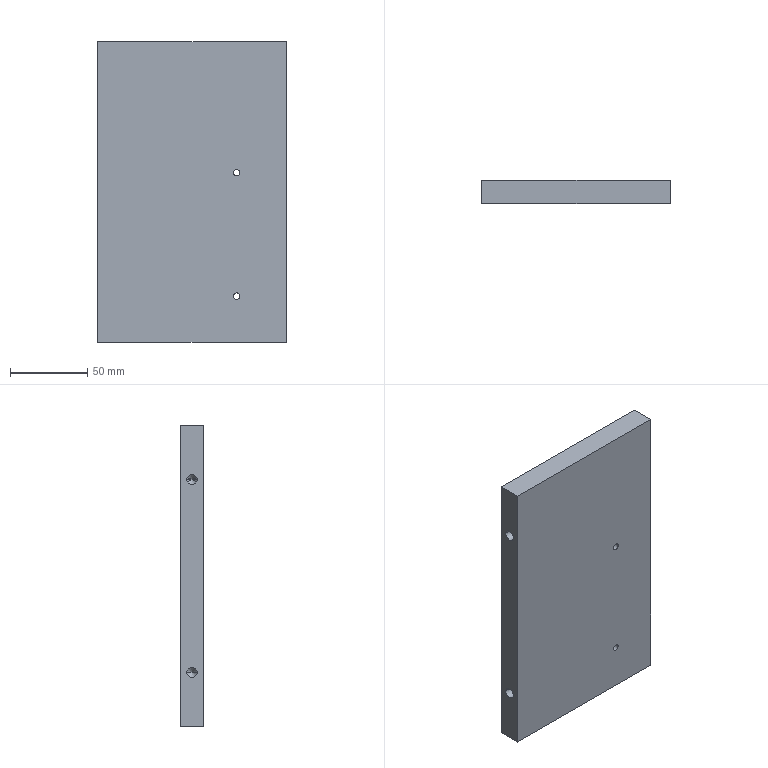Component | SolidWorks | InnerBagLiftingCylinderFixingPlate-1 | 1 solid | 26 faces | box 122 x 15 x 195 mm | volume 354555 mm3 | cylinder 12 | cone 8 | plane 6 | commonest cylinder face diameters 4.2 x8 6.8 x4
build123d program:
from build123d import *

# Parameters (mm, degrees)
SKETCH1_W             = 122
SKETCH1_H             = 195
BOSS_EXTRUDE1_DEPTH   = 7.5
M8_TAPPED_HOLE1_D     = 6.8
M8_TAPPED_HOLE1_DEPTH = 19.75
M8_TAPPED_HOLE1_TIP   = 3.4
M5_TAPPED_HOLE1_D     = 4.2
M5_TAPPED_HOLE2_D     = 4.2
M5_TAPPED_HOLE2_DEPTH = 12.4
M5_TAPPED_HOLE2_TIP   = 2.1


with BuildPart() as part:
    # Sketch1 → Boss-Extrude1 (new, symmetric)
    with BuildSketch(Plane.XY):
        with Locations((61, 97.5)):
            Rectangle(SKETCH1_W, SKETCH1_H)
    extrude(amount=BOSS_EXTRUDE1_DEPTH, both=True)

    # M8 Tapped Hole1
    with Locations(Plane(origin=(0, 160, 0), x_dir=(0, 0, -1), z_dir=(-1, 0, 0))):
        with Locations((0, 0), (0, 125)):
            Hole(M8_TAPPED_HOLE1_D / 2, depth=M8_TAPPED_HOLE1_DEPTH)
            with Locations((0, 0, -(M8_TAPPED_HOLE1_DEPTH + M8_TAPPED_HOLE1_TIP / 2))):  # 90° drill point
                Cone(0, M8_TAPPED_HOLE1_D / 2, M8_TAPPED_HOLE1_TIP, mode=Mode.SUBTRACT)

    # M5 Tapped Hole1 (through all)
    with Locations(Plane(origin=(90, 110, 7.5), x_dir=(1, 0, 0), z_dir=(0, 0, 1))):
        with Locations((0, 0), (0, -80)):
            Hole(M5_TAPPED_HOLE1_D / 2)

    # M5 Tapped Hole2
    with Locations(Plane(origin=(0, 0, 0), x_dir=(-1, 0, 0), z_dir=(0, -1, 0))):
        with Locations((-76, 0), (-104, 0)):
            Hole(M5_TAPPED_HOLE2_D / 2, depth=M5_TAPPED_HOLE2_DEPTH)
            with Locations((0, 0, -(M5_TAPPED_HOLE2_DEPTH + M5_TAPPED_HOLE2_TIP / 2))):  # 90° drill point
                Cone(0, M5_TAPPED_HOLE2_D / 2, M5_TAPPED_HOLE2_TIP, mode=Mode.SUBTRACT)


solid = part.part

# Placed as in the assembly
solid = solid.moved(Location((-22.646, -26.568, 148.933), (90, 0, 0)))
STEP:
#1=COLOUR_RGB('',0.7922,0.8196,0.9333);
#2=FILL_AREA_STYLE_COLOUR('',#1);
#3=FILL_AREA_STYLE('',(#2));
#4=SURFACE_STYLE_FILL_AREA(#3);
#5=SURFACE_SIDE_STYLE('',(#4));
#6=SURFACE_STYLE_USAGE(.BOTH.,#5);
#7=PRESENTATION_STYLE_ASSIGNMENT((#6));
#8=CARTESIAN_POINT('',(2.101,-1.129,6.352));
#9=VERTEX_POINT('',#8);
#10=CARTESIAN_POINT('',(2.101,-0.9633,6.352));
#11=VERTEX_POINT('',#10);
#12=CARTESIAN_POINT('',(2.101,-1.046,6.352));
#13=DIRECTION('',(0.,0.,-1.));
#14=DIRECTION('',(0.,1.,0.));
#15=AXIS2_PLACEMENT_3D('',#12,#13,#14);
#16=CIRCLE('',#15,0.08268);
#17=EDGE_CURVE('',#9,#11,#16,.T.);
#18=ORIENTED_EDGE('',*,*,#17,.F.);
#19=CARTESIAN_POINT('',(2.101,-1.129,5.863));
#20=VERTEX_POINT('',#19);
#21=CARTESIAN_POINT('',(2.101,-1.129,5.863));
#22=DIRECTION('',(0.,0.,-1.));
#23=VECTOR('',#22,39.37);
#24=LINE('',#21,#23);
#25=EDGE_CURVE('',#9,#20,#24,.T.);
#26=ORIENTED_EDGE('',*,*,#25,.T.);
#27=CARTESIAN_POINT('',(2.101,-0.9633,5.863));
#28=VERTEX_POINT('',#27);
#29=CARTESIAN_POINT('',(2.101,-1.046,5.863));
#30=DIRECTION('',(0.,0.,-1.));
#31=DIRECTION('',(0.,1.,0.));
#32=AXIS2_PLACEMENT_3D('',#29,#30,#31);
#33=CIRCLE('',#32,0.08268);
#34=EDGE_CURVE('',#20,#28,#33,.T.);
#35=ORIENTED_EDGE('',*,*,#34,.T.);
#36=CARTESIAN_POINT('',(2.101,-0.9633,5.863));
#37=DIRECTION('',(0.,0.,-1.));
#38=VECTOR('',#37,39.37);
#39=LINE('',#36,#38);
#40=EDGE_CURVE('',#11,#28,#39,.T.);
#41=ORIENTED_EDGE('',*,*,#40,.F.);
#42=EDGE_LOOP('',(#18,#26,#35,#41));
#43=FACE_OUTER_BOUND('',#42,.T.);
#44=CARTESIAN_POINT('',(2.101,-1.046,5.863));
#45=DIRECTION('',(0.,0.,-1.));
#46=DIRECTION('',(0.,1.,0.));
#47=AXIS2_PLACEMENT_3D('',#44,#45,#46);
#48=CYLINDRICAL_SURFACE('',#47,0.08268);
#49=ADVANCED_FACE('',(#43),#48,.F.);
#50=CARTESIAN_POINT('',(2.101,-1.046,6.434));
#51=VERTEX_POINT('',#50);
#52=CARTESIAN_POINT('',(2.101,-0.9633,6.352));
#53=DIRECTION('',(0.,0.7071,-0.7071));
#54=VECTOR('',#53,39.37);
#55=LINE('',#52,#54);
#56=EDGE_CURVE('',#51,#11,#55,.T.);
#57=ORIENTED_EDGE('',*,*,#56,.F.);
#58=CARTESIAN_POINT('',(2.101,-1.129,6.352));
#59=DIRECTION('',(0.,-0.7071,-0.7071));
#60=VECTOR('',#59,39.37);
#61=LINE('',#58,#60);
#62=EDGE_CURVE('',#51,#9,#61,.T.);
#63=ORIENTED_EDGE('',*,*,#62,.T.);
#64=ORIENTED_EDGE('',*,*,#17,.T.);
#65=EDGE_LOOP('',(#57,#63,#64));
#66=FACE_OUTER_BOUND('',#65,.T.);
#67=CARTESIAN_POINT('',(2.101,-1.046,6.352));
#68=DIRECTION('',(0.,0.,-1.));
#69=DIRECTION('',(0.,1.,0.));
#70=AXIS2_PLACEMENT_3D('',#67,#68,#69);
#71=CONICAL_SURFACE('',#70,0.08268,0.7854);
#72=ADVANCED_FACE('',(#66),#71,.F.);
#73=CARTESIAN_POINT('',(3.203,-1.129,6.352));
#74=VERTEX_POINT('',#73);
#75=CARTESIAN_POINT('',(3.203,-0.9633,6.352));
#76=VERTEX_POINT('',#75);
#77=CARTESIAN_POINT('',(3.203,-1.046,6.352));
#78=DIRECTION('',(0.,0.,-1.));
#79=DIRECTION('',(0.,1.,0.));
#80=AXIS2_PLACEMENT_3D('',#77,#78,#79);
#81=CIRCLE('',#80,0.08268);
#82=EDGE_CURVE('',#74,#76,#81,.T.);
#83=ORIENTED_EDGE('',*,*,#82,.F.);
#84=CARTESIAN_POINT('',(3.203,-1.129,5.863));
#85=VERTEX_POINT('',#84);
#86=CARTESIAN_POINT('',(3.203,-1.129,5.863));
#87=DIRECTION('',(0.,0.,-1.));
#88=VECTOR('',#87,39.37);
#89=LINE('',#86,#88);
#90=EDGE_CURVE('',#74,#85,#89,.T.);
#91=ORIENTED_EDGE('',*,*,#90,.T.);
#92=CARTESIAN_POINT('',(3.203,-0.9633,5.863));
#93=VERTEX_POINT('',#92);
#94=CARTESIAN_POINT('',(3.203,-1.046,5.863));
#95=DIRECTION('',(0.,0.,-1.));
#96=DIRECTION('',(0.,1.,0.));
#97=AXIS2_PLACEMENT_3D('',#94,#95,#96);
#98=CIRCLE('',#97,0.08268);
#99=EDGE_CURVE('',#85,#93,#98,.T.);
#100=ORIENTED_EDGE('',*,*,#99,.T.);
#101=CARTESIAN_POINT('',(3.203,-0.9633,5.863));
#102=DIRECTION('',(0.,0.,-1.));
#103=VECTOR('',#102,39.37);
#104=LINE('',#101,#103);
#105=EDGE_CURVE('',#76,#93,#104,.T.);
#106=ORIENTED_EDGE('',*,*,#105,.F.);
#107=EDGE_LOOP('',(#83,#91,#100,#106));
#108=FACE_OUTER_BOUND('',#107,.T.);
#109=CARTESIAN_POINT('',(3.203,-1.046,5.863));
#110=DIRECTION('',(0.,0.,-1.));
#111=DIRECTION('',(0.,1.,0.));
#112=AXIS2_PLACEMENT_3D('',#109,#110,#111);
#113=CYLINDRICAL_SURFACE('',#112,0.08268);
#114=ADVANCED_FACE('',(#108),#113,.F.);
#115=CARTESIAN_POINT('',(3.203,-1.046,6.434));
#116=VERTEX_POINT('',#115);
#117=CARTESIAN_POINT('',(3.203,-0.9633,6.352));
#118=DIRECTION('',(0.,0.7071,-0.7071));
#119=VECTOR('',#118,39.37);
#120=LINE('',#117,#119);
#121=EDGE_CURVE('',#116,#76,#120,.T.);
#122=ORIENTED_EDGE('',*,*,#121,.F.);
#123=CARTESIAN_POINT('',(3.203,-1.129,6.352));
#124=DIRECTION('',(0.,-0.7071,-0.7071));
#125=VECTOR('',#124,39.37);
#126=LINE('',#123,#125);
#127=EDGE_CURVE('',#116,#74,#126,.T.);
#128=ORIENTED_EDGE('',*,*,#127,.T.);
#129=ORIENTED_EDGE('',*,*,#82,.T.);
#130=EDGE_LOOP('',(#122,#128,#129));
#131=FACE_OUTER_BOUND('',#130,.T.);
#132=CARTESIAN_POINT('',(3.203,-1.046,6.352));
#133=DIRECTION('',(0.,0.,-1.));
#134=DIRECTION('',(0.,1.,0.));
#135=AXIS2_PLACEMENT_3D('',#132,#133,#134);
#136=CONICAL_SURFACE('',#135,0.08268,0.7854);
#137=ADVANCED_FACE('',(#131),#136,.F.);
#138=CARTESIAN_POINT('',(2.569,-0.7507,10.194));
#139=VERTEX_POINT('',#138);
#140=CARTESIAN_POINT('',(2.734,-0.7507,10.194));
#141=VERTEX_POINT('',#140);
#142=CARTESIAN_POINT('',(2.652,-0.7507,10.194));
#143=DIRECTION('',(0.,-1.,0.));
#144=DIRECTION('',(1.,0.,0.));
#145=AXIS2_PLACEMENT_3D('',#142,#143,#144);
#146=CIRCLE('',#145,0.08268);
#147=EDGE_CURVE('',#139,#141,#146,.T.);
#148=ORIENTED_EDGE('',*,*,#147,.F.);
#149=CARTESIAN_POINT('',(2.569,-1.341,10.194));
#150=VERTEX_POINT('',#149);
#151=CARTESIAN_POINT('',(2.569,-1.341,10.194));
#152=DIRECTION('',(0.,-1.,0.));
#153=VECTOR('',#152,39.37);
#154=LINE('',#151,#153);
#155=EDGE_CURVE('',#139,#150,#154,.T.);
#156=ORIENTED_EDGE('',*,*,#155,.T.);
#157=CARTESIAN_POINT('',(2.734,-1.341,10.194));
#158=VERTEX_POINT('',#157);
#159=CARTESIAN_POINT('',(2.652,-1.341,10.194));
#160=DIRECTION('',(0.,-1.,0.));
#161=DIRECTION('',(1.,0.,0.));
#162=AXIS2_PLACEMENT_3D('',#159,#160,#161);
#163=CIRCLE('',#162,0.08268);
#164=EDGE_CURVE('',#150,#158,#163,.T.);
#165=ORIENTED_EDGE('',*,*,#164,.T.);
#166=CARTESIAN_POINT('',(2.734,-1.341,10.194));
#167=DIRECTION('',(0.,-1.,0.));
#168=VECTOR('',#167,39.37);
#169=LINE('',#166,#168);
#170=EDGE_CURVE('',#141,#158,#169,.T.);
#171=ORIENTED_EDGE('',*,*,#170,.F.);
#172=EDGE_LOOP('',(#148,#156,#165,#171));
#173=FACE_OUTER_BOUND('',#172,.T.);
#174=CARTESIAN_POINT('',(2.652,-1.341,10.194));
#175=DIRECTION('',(0.,-1.,0.));
#176=DIRECTION('',(1.,0.,0.));
#177=AXIS2_PLACEMENT_3D('',#174,#175,#176);
#178=CYLINDRICAL_SURFACE('',#177,0.08268);
#179=ADVANCED_FACE('',(#173),#178,.F.);
#180=CARTESIAN_POINT('',(2.569,-0.7507,7.045));
#181=VERTEX_POINT('',#180);
#182=CARTESIAN_POINT('',(2.734,-0.7507,7.045));
#183=VERTEX_POINT('',#182);
#184=CARTESIAN_POINT('',(2.652,-0.7507,7.045));
#185=DIRECTION('',(0.,-1.,0.));
#186=DIRECTION('',(1.,0.,0.));
#187=AXIS2_PLACEMENT_3D('',#184,#185,#186);
#188=CIRCLE('',#187,0.08268);
#189=EDGE_CURVE('',#181,#183,#188,.T.);
#190=ORIENTED_EDGE('',*,*,#189,.F.);
#191=CARTESIAN_POINT('',(2.569,-1.341,7.045));
#192=VERTEX_POINT('',#191);
#193=CARTESIAN_POINT('',(2.569,-1.341,7.045));
#194=DIRECTION('',(0.,-1.,0.));
#195=VECTOR('',#194,39.37);
#196=LINE('',#193,#195);
#197=EDGE_CURVE('',#181,#192,#196,.T.);
#198=ORIENTED_EDGE('',*,*,#197,.T.);
#199=CARTESIAN_POINT('',(2.734,-1.341,7.045));
#200=VERTEX_POINT('',#199);
#201=CARTESIAN_POINT('',(2.652,-1.341,7.045));
#202=DIRECTION('',(0.,-1.,0.));
#203=DIRECTION('',(1.,0.,0.));
#204=AXIS2_PLACEMENT_3D('',#201,#202,#203);
#205=CIRCLE('',#204,0.08268);
#206=EDGE_CURVE('',#192,#200,#205,.T.);
#207=ORIENTED_EDGE('',*,*,#206,.T.);
#208=CARTESIAN_POINT('',(2.734,-1.341,7.045));
#209=DIRECTION('',(0.,-1.,0.));
#210=VECTOR('',#209,39.37);
#211=LINE('',#208,#210);
#212=EDGE_CURVE('',#183,#200,#211,.T.);
#213=ORIENTED_EDGE('',*,*,#212,.F.);
#214=EDGE_LOOP('',(#190,#198,#207,#213));
#215=FACE_OUTER_BOUND('',#214,.T.);
#216=CARTESIAN_POINT('',(2.652,-1.341,7.045));
#217=DIRECTION('',(0.,-1.,0.));
#218=DIRECTION('',(1.,0.,0.));
#219=AXIS2_PLACEMENT_3D('',#216,#217,#218);
#220=CYLINDRICAL_SURFACE('',#219,0.08268);
#221=ADVANCED_FACE('',(#215),#220,.F.);
#222=CARTESIAN_POINT('',(-0.114,-0.9121,12.163));
#223=VERTEX_POINT('',#222);
#224=CARTESIAN_POINT('',(-0.114,-1.18,12.163));
#225=VERTEX_POINT('',#224);
#226=CARTESIAN_POINT('',(-0.114,-1.046,12.163));
#227=DIRECTION('',(-1.,0.,0.));
#228=DIRECTION('',(0.,-1.,0.));
#229=AXIS2_PLACEMENT_3D('',#226,#227,#228);
#230=CIRCLE('',#229,0.1339);
#231=EDGE_CURVE('',#223,#225,#230,.T.);
#232=ORIENTED_EDGE('',*,*,#231,.F.);
#233=CARTESIAN_POINT('',(-0.8916,-0.9121,12.163));
#234=VERTEX_POINT('',#233);
#235=CARTESIAN_POINT('',(-0.8916,-0.9121,12.163));
#236=DIRECTION('',(-1.,0.,0.));
#237=VECTOR('',#236,39.37);
#238=LINE('',#235,#237);
#239=EDGE_CURVE('',#223,#234,#238,.T.);
#240=ORIENTED_EDGE('',*,*,#239,.T.);
#241=CARTESIAN_POINT('',(-0.8916,-1.18,12.163));
#242=VERTEX_POINT('',#241);
#243=CARTESIAN_POINT('',(-0.8916,-1.046,12.163));
#244=DIRECTION('',(-1.,0.,0.));
#245=DIRECTION('',(0.,-1.,0.));
#246=AXIS2_PLACEMENT_3D('',#243,#244,#245);
#247=CIRCLE('',#246,0.1339);
#248=EDGE_CURVE('',#234,#242,#247,.T.);
#249=ORIENTED_EDGE('',*,*,#248,.T.);
#250=CARTESIAN_POINT('',(-0.8916,-1.18,12.163));
#251=DIRECTION('',(-1.,0.,0.));
#252=VECTOR('',#251,39.37);
#253=LINE('',#250,#252);
#254=EDGE_CURVE('',#225,#242,#253,.T.);
#255=ORIENTED_EDGE('',*,*,#254,.F.);
#256=EDGE_LOOP('',(#232,#240,#249,#255));
#257=FACE_OUTER_BOUND('',#256,.T.);
#258=CARTESIAN_POINT('',(-0.8916,-1.046,12.163));
#259=DIRECTION('',(-1.,0.,0.));
#260=DIRECTION('',(0.,-1.,0.));
#261=AXIS2_PLACEMENT_3D('',#258,#259,#260);
#262=CYLINDRICAL_SURFACE('',#261,0.1339);
#263=ADVANCED_FACE('',(#257),#262,.F.);
#264=CARTESIAN_POINT('',(0.01983,-1.046,12.163));
#265=VERTEX_POINT('',#264);
#266=CARTESIAN_POINT('',(-0.114,-1.18,12.163));
#267=DIRECTION('',(-0.7071,-0.7071,0.));
#268=VECTOR('',#267,39.37);
#269=LINE('',#266,#268);
#270=EDGE_CURVE('',#265,#225,#269,.T.);
#271=ORIENTED_EDGE('',*,*,#270,.F.);
#272=CARTESIAN_POINT('',(-0.114,-0.9121,12.163));
#273=DIRECTION('',(-0.7071,0.7071,0.));
#274=VECTOR('',#273,39.37);
#275=LINE('',#272,#274);
#276=EDGE_CURVE('',#265,#223,#275,.T.);
#277=ORIENTED_EDGE('',*,*,#276,.T.);
#278=ORIENTED_EDGE('',*,*,#231,.T.);
#279=EDGE_LOOP('',(#271,#277,#278));
#280=FACE_OUTER_BOUND('',#279,.T.);
#281=CARTESIAN_POINT('',(-0.114,-1.046,12.163));
#282=DIRECTION('',(-1.,0.,0.));
#283=DIRECTION('',(0.,-1.,0.));
#284=AXIS2_PLACEMENT_3D('',#281,#282,#283);
#285=CONICAL_SURFACE('',#284,0.1339,0.7854);
#286=ADVANCED_FACE('',(#280),#285,.F.);
#287=CARTESIAN_POINT('',(-0.114,-0.9121,7.241));
#288=VERTEX_POINT('',#287);
#289=CARTESIAN_POINT('',(-0.114,-1.18,7.241));
#290=VERTEX_POINT('',#289);
#291=CARTESIAN_POINT('',(-0.114,-1.046,7.241));
#292=DIRECTION('',(-1.,0.,0.));
#293=DIRECTION('',(0.,-1.,0.));
#294=AXIS2_PLACEMENT_3D('',#291,#292,#293);
#295=CIRCLE('',#294,0.1339);
#296=EDGE_CURVE('',#288,#290,#295,.T.);
#297=ORIENTED_EDGE('',*,*,#296,.F.);
#298=CARTESIAN_POINT('',(-0.8916,-0.9121,7.241));
#299=VERTEX_POINT('',#298);
#300=CARTESIAN_POINT('',(-0.8916,-0.9121,7.241));
#301=DIRECTION('',(-1.,0.,0.));
#302=VECTOR('',#301,39.37);
#303=LINE('',#300,#302);
#304=EDGE_CURVE('',#288,#299,#303,.T.);
#305=ORIENTED_EDGE('',*,*,#304,.T.);
#306=CARTESIAN_POINT('',(-0.8916,-1.18,7.241));
#307=VERTEX_POINT('',#306);
#308=CARTESIAN_POINT('',(-0.8916,-1.046,7.241));
#309=DIRECTION('',(-1.,0.,0.));
#310=DIRECTION('',(0.,-1.,0.));
#311=AXIS2_PLACEMENT_3D('',#308,#309,#310);
#312=CIRCLE('',#311,0.1339);
#313=EDGE_CURVE('',#299,#307,#312,.T.);
#314=ORIENTED_EDGE('',*,*,#313,.T.);
#315=CARTESIAN_POINT('',(-0.8916,-1.18,7.241));
#316=DIRECTION('',(-1.,0.,0.));
#317=VECTOR('',#316,39.37);
#318=LINE('',#315,#317);
#319=EDGE_CURVE('',#290,#307,#318,.T.);
#320=ORIENTED_EDGE('',*,*,#319,.F.);
#321=EDGE_LOOP('',(#297,#305,#314,#320));
#322=FACE_OUTER_BOUND('',#321,.T.);
#323=CARTESIAN_POINT('',(-0.8916,-1.046,7.241));
#324=DIRECTION('',(-1.,0.,0.));
#325=DIRECTION('',(0.,-1.,0.));
#326=AXIS2_PLACEMENT_3D('',#323,#324,#325);
#327=CYLINDRICAL_SURFACE('',#326,0.1339);
#328=ADVANCED_FACE('',(#322),#327,.F.);
#329=CARTESIAN_POINT('',(0.01983,-1.046,7.241));
#330=VERTEX_POINT('',#329);
#331=CARTESIAN_POINT('',(-0.114,-1.18,7.241));
#332=DIRECTION('',(-0.7071,-0.7071,0.));
#333=VECTOR('',#332,39.37);
#334=LINE('',#331,#333);
#335=EDGE_CURVE('',#330,#290,#334,.T.);
#336=ORIENTED_EDGE('',*,*,#335,.F.);
#337=CARTESIAN_POINT('',(-0.114,-0.9121,7.241));
#338=DIRECTION('',(-0.7071,0.7071,0.));
#339=VECTOR('',#338,39.37);
#340=LINE('',#337,#339);
#341=EDGE_CURVE('',#330,#288,#340,.T.);
#342=ORIENTED_EDGE('',*,*,#341,.T.);
#343=ORIENTED_EDGE('',*,*,#296,.T.);
#344=EDGE_LOOP('',(#336,#342,#343));
#345=FACE_OUTER_BOUND('',#344,.T.);
#346=CARTESIAN_POINT('',(-0.114,-1.046,7.241));
#347=DIRECTION('',(-1.,0.,0.));
#348=DIRECTION('',(0.,-1.,0.));
#349=AXIS2_PLACEMENT_3D('',#346,#347,#348);
#350=CONICAL_SURFACE('',#349,0.1339,0.7854);
#351=ADVANCED_FACE('',(#345),#350,.F.);
#352=CARTESIAN_POINT('',(2.652,-1.341,10.194));
#353=DIRECTION('',(0.,-1.,0.));
#354=DIRECTION('',(1.,0.,0.));
#355=AXIS2_PLACEMENT_3D('',#352,#353,#354);
#356=CIRCLE('',#355,0.08268);
#357=EDGE_CURVE('',#158,#150,#356,.T.);
#358=ORIENTED_EDGE('',*,*,#357,.F.);
#359=ORIENTED_EDGE('',*,*,#164,.F.);
#360=EDGE_LOOP('',(#358,#359));
#361=FACE_BOUND('',#360,.T.);
#362=CARTESIAN_POINT('',(-0.8916,-1.341,13.541));
#363=VERTEX_POINT('',#362);
#364=CARTESIAN_POINT('',(-0.8916,-1.341,5.863));
#365=VERTEX_POINT('',#364);
#366=CARTESIAN_POINT('',(-0.8916,-1.341,5.863));
#367=DIRECTION('',(0.,0.,-1.));
#368=VECTOR('',#367,39.37);
#369=LINE('',#366,#368);
#370=EDGE_CURVE('',#363,#365,#369,.T.);
#371=ORIENTED_EDGE('',*,*,#370,.T.);
#372=CARTESIAN_POINT('',(3.912,-1.341,5.863));
#373=VERTEX_POINT('',#372);
#374=CARTESIAN_POINT('',(-0.8916,-1.341,5.863));
#375=DIRECTION('',(1.,0.,0.));
#376=VECTOR('',#375,39.37);
#377=LINE('',#374,#376);
#378=EDGE_CURVE('',#365,#373,#377,.T.);
#379=ORIENTED_EDGE('',*,*,#378,.T.);
#380=CARTESIAN_POINT('',(3.912,-1.341,13.541));
#381=VERTEX_POINT('',#380);
#382=CARTESIAN_POINT('',(3.912,-1.341,5.863));
#383=DIRECTION('',(-0.,0.,1.));
#384=VECTOR('',#383,39.37);
#385=LINE('',#382,#384);
#386=EDGE_CURVE('',#373,#381,#385,.T.);
#387=ORIENTED_EDGE('',*,*,#386,.T.);
#388=CARTESIAN_POINT('',(-0.8916,-1.341,13.541));
#389=DIRECTION('',(-1.,0.,0.));
#390=VECTOR('',#389,39.37);
#391=LINE('',#388,#390);
#392=EDGE_CURVE('',#381,#363,#391,.T.);
#393=ORIENTED_EDGE('',*,*,#392,.T.);
#394=EDGE_LOOP('',(#371,#379,#387,#393));
#395=FACE_OUTER_BOUND('',#394,.T.);
#396=CARTESIAN_POINT('',(2.652,-1.341,7.045));
#397=DIRECTION('',(0.,-1.,0.));
#398=DIRECTION('',(1.,0.,0.));
#399=AXIS2_PLACEMENT_3D('',#396,#397,#398);
#400=CIRCLE('',#399,0.08268);
#401=EDGE_CURVE('',#200,#192,#400,.T.);
#402=ORIENTED_EDGE('',*,*,#401,.F.);
#403=ORIENTED_EDGE('',*,*,#206,.F.);
#404=EDGE_LOOP('',(#402,#403));
#405=FACE_BOUND('',#404,.T.);
#406=CARTESIAN_POINT('',(-0.8916,-1.341,5.863));
#407=DIRECTION('',(0.,1.,0.));
#408=DIRECTION('',(-1.,0.,0.));
#409=AXIS2_PLACEMENT_3D('',#406,#407,#408);
#410=PLANE('',#409);
#411=ADVANCED_FACE('',(#361,#395,#405),#410,.F.);
#412=CARTESIAN_POINT('',(-0.8916,-1.046,12.163));
#413=DIRECTION('',(-1.,0.,0.));
#414=DIRECTION('',(0.,-1.,0.));
#415=AXIS2_PLACEMENT_3D('',#412,#413,#414);
#416=CIRCLE('',#415,0.1339);
#417=EDGE_CURVE('',#242,#234,#416,.T.);
#418=ORIENTED_EDGE('',*,*,#417,.F.);
#419=ORIENTED_EDGE('',*,*,#248,.F.);
#420=EDGE_LOOP('',(#418,#419));
#421=FACE_BOUND('',#420,.T.);
#422=CARTESIAN_POINT('',(-0.8916,-1.046,7.241));
#423=DIRECTION('',(-1.,0.,0.));
#424=DIRECTION('',(0.,-1.,0.));
#425=AXIS2_PLACEMENT_3D('',#422,#423,#424);
#426=CIRCLE('',#425,0.1339);
#427=EDGE_CURVE('',#307,#299,#426,.T.);
#428=ORIENTED_EDGE('',*,*,#427,.F.);
#429=ORIENTED_EDGE('',*,*,#313,.F.);
#430=EDGE_LOOP('',(#428,#429));
#431=FACE_BOUND('',#430,.T.);
#432=CARTESIAN_POINT('',(-0.8916,-0.7507,13.541));
#433=VERTEX_POINT('',#432);
#434=CARTESIAN_POINT('',(-0.8916,-0.7507,5.863));
#435=VERTEX_POINT('',#434);
#436=CARTESIAN_POINT('',(-0.8916,-0.7507,5.863));
#437=DIRECTION('',(0.,0.,-1.));
#438=VECTOR('',#437,39.37);
#439=LINE('',#436,#438);
#440=EDGE_CURVE('',#433,#435,#439,.T.);
#441=ORIENTED_EDGE('',*,*,#440,.T.);
#442=CARTESIAN_POINT('',(-0.8916,-1.341,5.863));
#443=DIRECTION('',(0.,1.,0.));
#444=VECTOR('',#443,39.37);
#445=LINE('',#442,#444);
#446=EDGE_CURVE('',#365,#435,#445,.T.);
#447=ORIENTED_EDGE('',*,*,#446,.F.);
#448=ORIENTED_EDGE('',*,*,#370,.F.);
#449=CARTESIAN_POINT('',(-0.8916,-1.341,13.541));
#450=DIRECTION('',(0.,1.,0.));
#451=VECTOR('',#450,39.37);
#452=LINE('',#449,#451);
#453=EDGE_CURVE('',#363,#433,#452,.T.);
#454=ORIENTED_EDGE('',*,*,#453,.T.);
#455=EDGE_LOOP('',(#441,#447,#448,#454));
#456=FACE_OUTER_BOUND('',#455,.T.);
#457=CARTESIAN_POINT('',(-0.8916,-1.341,5.863));
#458=DIRECTION('',(1.,0.,0.));
#459=DIRECTION('',(0.,1.,0.));
#460=AXIS2_PLACEMENT_3D('',#457,#458,#459);
#461=PLANE('',#460);
#462=ADVANCED_FACE('',(#421,#431,#456),#461,.F.);
#463=CARTESIAN_POINT('',(2.101,-1.046,5.863));
#464=DIRECTION('',(0.,0.,-1.));
#465=DIRECTION('',(0.,1.,0.));
#466=AXIS2_PLACEMENT_3D('',#463,#464,#465);
#467=CIRCLE('',#466,0.08268);
#468=EDGE_CURVE('',#28,#20,#467,.T.);
#469=ORIENTED_EDGE('',*,*,#468,.F.);
#470=ORIENTED_EDGE('',*,*,#34,.F.);
#471=EDGE_LOOP('',(#469,#470));
#472=FACE_BOUND('',#471,.T.);
#473=CARTESIAN_POINT('',(3.203,-1.046,5.863));
#474=DIRECTION('',(0.,0.,-1.));
#475=DIRECTION('',(0.,1.,0.));
#476=AXIS2_PLACEMENT_3D('',#473,#474,#475);
#477=CIRCLE('',#476,0.08268);
#478=EDGE_CURVE('',#93,#85,#477,.T.);
#479=ORIENTED_EDGE('',*,*,#478,.F.);
#480=ORIENTED_EDGE('',*,*,#99,.F.);
#481=EDGE_LOOP('',(#479,#480));
#482=FACE_BOUND('',#481,.T.);
#483=CARTESIAN_POINT('',(3.912,-0.7507,5.863));
#484=VERTEX_POINT('',#483);
#485=CARTESIAN_POINT('',(-0.8916,-0.7507,5.863));
#486=DIRECTION('',(1.,0.,0.));
#487=VECTOR('',#486,39.37);
#488=LINE('',#485,#487);
#489=EDGE_CURVE('',#435,#484,#488,.T.);
#490=ORIENTED_EDGE('',*,*,#489,.T.);
#491=CARTESIAN_POINT('',(3.912,-1.341,5.863));
#492=DIRECTION('',(0.,1.,0.));
#493=VECTOR('',#492,39.37);
#494=LINE('',#491,#493);
#495=EDGE_CURVE('',#373,#484,#494,.T.);
#496=ORIENTED_EDGE('',*,*,#495,.F.);
#497=ORIENTED_EDGE('',*,*,#378,.F.);
#498=ORIENTED_EDGE('',*,*,#446,.T.);
#499=EDGE_LOOP('',(#490,#496,#497,#498));
#500=FACE_OUTER_BOUND('',#499,.T.);
#501=CARTESIAN_POINT('',(-0.8916,-1.341,5.863));
#502=DIRECTION('',(0.,0.,1.));
#503=DIRECTION('',(0.,-1.,0.));
#504=AXIS2_PLACEMENT_3D('',#501,#502,#503);
#505=PLANE('',#504);
#506=ADVANCED_FACE('',(#472,#482,#500),#505,.F.);
#507=CARTESIAN_POINT('',(3.912,-0.7507,13.541));
#508=VERTEX_POINT('',#507);
#509=CARTESIAN_POINT('',(3.912,-0.7507,5.863));
#510=DIRECTION('',(-0.,0.,1.));
#511=VECTOR('',#510,39.37);
#512=LINE('',#509,#511);
#513=EDGE_CURVE('',#484,#508,#512,.T.);
#514=ORIENTED_EDGE('',*,*,#513,.T.);
#515=CARTESIAN_POINT('',(3.912,-1.341,13.541));
#516=DIRECTION('',(0.,1.,0.));
#517=VECTOR('',#516,39.37);
#518=LINE('',#515,#517);
#519=EDGE_CURVE('',#381,#508,#518,.T.);
#520=ORIENTED_EDGE('',*,*,#519,.F.);
#521=ORIENTED_EDGE('',*,*,#386,.F.);
#522=ORIENTED_EDGE('',*,*,#495,.T.);
#523=EDGE_LOOP('',(#514,#520,#521,#522));
#524=FACE_OUTER_BOUND('',#523,.T.);
#525=CARTESIAN_POINT('',(3.912,-1.341,5.863));
#526=DIRECTION('',(-1.,0.,-0.));
#527=DIRECTION('',(0.,0.,-1.));
#528=AXIS2_PLACEMENT_3D('',#525,#526,#527);
#529=PLANE('',#528);
#530=ADVANCED_FACE('',(#524),#529,.F.);
#531=CARTESIAN_POINT('',(-0.8916,-0.7507,13.541));
#532=DIRECTION('',(-1.,0.,0.));
#533=VECTOR('',#532,39.37);
#534=LINE('',#531,#533);
#535=EDGE_CURVE('',#508,#433,#534,.T.);
#536=ORIENTED_EDGE('',*,*,#535,.T.);
#537=ORIENTED_EDGE('',*,*,#453,.F.);
#538=ORIENTED_EDGE('',*,*,#392,.F.);
#539=ORIENTED_EDGE('',*,*,#519,.T.);
#540=EDGE_LOOP('',(#536,#537,#538,#539));
#541=FACE_OUTER_BOUND('',#540,.T.);
#542=CARTESIAN_POINT('',(-0.8916,-1.341,13.541));
#543=DIRECTION('',(0.,0.,-1.));
#544=DIRECTION('',(0.,1.,0.));
#545=AXIS2_PLACEMENT_3D('',#542,#543,#544);
#546=PLANE('',#545);
#547=ADVANCED_FACE('',(#541),#546,.F.);
#548=CARTESIAN_POINT('',(2.652,-0.7507,10.194));
#549=DIRECTION('',(0.,-1.,0.));
#550=DIRECTION('',(1.,0.,0.));
#551=AXIS2_PLACEMENT_3D('',#548,#549,#550);
#552=CIRCLE('',#551,0.08268);
#553=EDGE_CURVE('',#141,#139,#552,.T.);
#554=ORIENTED_EDGE('',*,*,#553,.T.);
#555=ORIENTED_EDGE('',*,*,#147,.T.);
#556=EDGE_LOOP('',(#554,#555));
#557=FACE_BOUND('',#556,.T.);
#558=CARTESIAN_POINT('',(2.652,-0.7507,7.045));
#559=DIRECTION('',(0.,-1.,0.));
#560=DIRECTION('',(1.,0.,0.));
#561=AXIS2_PLACEMENT_3D('',#558,#559,#560);
#562=CIRCLE('',#561,0.08268);
#563=EDGE_CURVE('',#183,#181,#562,.T.);
#564=ORIENTED_EDGE('',*,*,#563,.T.);
#565=ORIENTED_EDGE('',*,*,#189,.T.);
#566=EDGE_LOOP('',(#564,#565));
#567=FACE_BOUND('',#566,.T.);
#568=ORIENTED_EDGE('',*,*,#440,.F.);
#569=ORIENTED_EDGE('',*,*,#535,.F.);
#570=ORIENTED_EDGE('',*,*,#513,.F.);
#571=ORIENTED_EDGE('',*,*,#489,.F.);
#572=EDGE_LOOP('',(#568,#569,#570,#571));
#573=FACE_OUTER_BOUND('',#572,.T.);
#574=CARTESIAN_POINT('',(-0.8916,-0.7507,5.863));
#575=DIRECTION('',(0.,1.,0.));
#576=DIRECTION('',(-1.,0.,0.));
#577=AXIS2_PLACEMENT_3D('',#574,#575,#576);
#578=PLANE('',#577);
#579=ADVANCED_FACE('',(#557,#567,#573),#578,.T.);
#580=ORIENTED_EDGE('',*,*,#341,.F.);
#581=ORIENTED_EDGE('',*,*,#335,.T.);
#582=CARTESIAN_POINT('',(-0.114,-1.046,7.241));
#583=DIRECTION('',(-1.,0.,0.));
#584=DIRECTION('',(0.,-1.,0.));
#585=AXIS2_PLACEMENT_3D('',#582,#583,#584);
#586=CIRCLE('',#585,0.1339);
#587=EDGE_CURVE('',#290,#288,#586,.T.);
#588=ORIENTED_EDGE('',*,*,#587,.T.);
#589=EDGE_LOOP('',(#580,#581,#588));
#590=FACE_OUTER_BOUND('',#589,.T.);
#591=CARTESIAN_POINT('',(-0.114,-1.046,7.241));
#592=DIRECTION('',(-1.,0.,0.));
#593=DIRECTION('',(0.,-1.,0.));
#594=AXIS2_PLACEMENT_3D('',#591,#592,#593);
#595=CONICAL_SURFACE('',#594,0.1339,0.7854);
#596=ADVANCED_FACE('',(#590),#595,.F.);
#597=ORIENTED_EDGE('',*,*,#304,.F.);
#598=ORIENTED_EDGE('',*,*,#587,.F.);
#599=ORIENTED_EDGE('',*,*,#319,.T.);
#600=ORIENTED_EDGE('',*,*,#427,.T.);
#601=EDGE_LOOP('',(#597,#598,#599,#600));
#602=FACE_OUTER_BOUND('',#601,.T.);
#603=CARTESIAN_POINT('',(-0.8916,-1.046,7.241));
#604=DIRECTION('',(-1.,0.,0.));
#605=DIRECTION('',(0.,-1.,0.));
#606=AXIS2_PLACEMENT_3D('',#603,#604,#605);
#607=CYLINDRICAL_SURFACE('',#606,0.1339);
#608=ADVANCED_FACE('',(#602),#607,.F.);
#609=ORIENTED_EDGE('',*,*,#276,.F.);
#610=ORIENTED_EDGE('',*,*,#270,.T.);
#611=CARTESIAN_POINT('',(-0.114,-1.046,12.163));
#612=DIRECTION('',(-1.,0.,0.));
#613=DIRECTION('',(0.,-1.,0.));
#614=AXIS2_PLACEMENT_3D('',#611,#612,#613);
#615=CIRCLE('',#614,0.1339);
#616=EDGE_CURVE('',#225,#223,#615,.T.);
#617=ORIENTED_EDGE('',*,*,#616,.T.);
#618=EDGE_LOOP('',(#609,#610,#617));
#619=FACE_OUTER_BOUND('',#618,.T.);
#620=CARTESIAN_POINT('',(-0.114,-1.046,12.163));
#621=DIRECTION('',(-1.,0.,0.));
#622=DIRECTION('',(0.,-1.,0.));
#623=AXIS2_PLACEMENT_3D('',#620,#621,#622);
#624=CONICAL_SURFACE('',#623,0.1339,0.7854);
#625=ADVANCED_FACE('',(#619),#624,.F.);
#626=ORIENTED_EDGE('',*,*,#239,.F.);
#627=ORIENTED_EDGE('',*,*,#616,.F.);
#628=ORIENTED_EDGE('',*,*,#254,.T.);
#629=ORIENTED_EDGE('',*,*,#417,.T.);
#630=EDGE_LOOP('',(#626,#627,#628,#629));
#631=FACE_OUTER_BOUND('',#630,.T.);
#632=CARTESIAN_POINT('',(-0.8916,-1.046,12.163));
#633=DIRECTION('',(-1.,0.,0.));
#634=DIRECTION('',(0.,-1.,0.));
#635=AXIS2_PLACEMENT_3D('',#632,#633,#634);
#636=CYLINDRICAL_SURFACE('',#635,0.1339);
#637=ADVANCED_FACE('',(#631),#636,.F.);
#638=ORIENTED_EDGE('',*,*,#197,.F.);
#639=ORIENTED_EDGE('',*,*,#563,.F.);
#640=ORIENTED_EDGE('',*,*,#212,.T.);
#641=ORIENTED_EDGE('',*,*,#401,.T.);
#642=EDGE_LOOP('',(#638,#639,#640,#641));
#643=FACE_OUTER_BOUND('',#642,.T.);
#644=CARTESIAN_POINT('',(2.652,-1.341,7.045));
#645=DIRECTION('',(0.,-1.,0.));
#646=DIRECTION('',(1.,0.,0.));
#647=AXIS2_PLACEMENT_3D('',#644,#645,#646);
#648=CYLINDRICAL_SURFACE('',#647,0.08268);
#649=ADVANCED_FACE('',(#643),#648,.F.);
#650=ORIENTED_EDGE('',*,*,#155,.F.);
#651=ORIENTED_EDGE('',*,*,#553,.F.);
#652=ORIENTED_EDGE('',*,*,#170,.T.);
#653=ORIENTED_EDGE('',*,*,#357,.T.);
#654=EDGE_LOOP('',(#650,#651,#652,#653));
#655=FACE_OUTER_BOUND('',#654,.T.);
#656=CARTESIAN_POINT('',(2.652,-1.341,10.194));
#657=DIRECTION('',(0.,-1.,0.));
#658=DIRECTION('',(1.,0.,0.));
#659=AXIS2_PLACEMENT_3D('',#656,#657,#658);
#660=CYLINDRICAL_SURFACE('',#659,0.08268);
#661=ADVANCED_FACE('',(#655),#660,.F.);
#662=ORIENTED_EDGE('',*,*,#127,.F.);
#663=ORIENTED_EDGE('',*,*,#121,.T.);
#664=CARTESIAN_POINT('',(3.203,-1.046,6.352));
#665=DIRECTION('',(0.,0.,-1.));
#666=DIRECTION('',(0.,1.,0.));
#667=AXIS2_PLACEMENT_3D('',#664,#665,#666);
#668=CIRCLE('',#667,0.08268);
#669=EDGE_CURVE('',#76,#74,#668,.T.);
#670=ORIENTED_EDGE('',*,*,#669,.T.);
#671=EDGE_LOOP('',(#662,#663,#670));
#672=FACE_OUTER_BOUND('',#671,.T.);
#673=CARTESIAN_POINT('',(3.203,-1.046,6.352));
#674=DIRECTION('',(0.,0.,-1.));
#675=DIRECTION('',(0.,1.,0.));
#676=AXIS2_PLACEMENT_3D('',#673,#674,#675);
#677=CONICAL_SURFACE('',#676,0.08268,0.7854);
#678=ADVANCED_FACE('',(#672),#677,.F.);
#679=ORIENTED_EDGE('',*,*,#90,.F.);
#680=ORIENTED_EDGE('',*,*,#669,.F.);
#681=ORIENTED_EDGE('',*,*,#105,.T.);
#682=ORIENTED_EDGE('',*,*,#478,.T.);
#683=EDGE_LOOP('',(#679,#680,#681,#682));
#684=FACE_OUTER_BOUND('',#683,.T.);
#685=CARTESIAN_POINT('',(3.203,-1.046,5.863));
#686=DIRECTION('',(0.,0.,-1.));
#687=DIRECTION('',(0.,1.,0.));
#688=AXIS2_PLACEMENT_3D('',#685,#686,#687);
#689=CYLINDRICAL_SURFACE('',#688,0.08268);
#690=ADVANCED_FACE('',(#684),#689,.F.);
#691=ORIENTED_EDGE('',*,*,#62,.F.);
#692=ORIENTED_EDGE('',*,*,#56,.T.);
#693=CARTESIAN_POINT('',(2.101,-1.046,6.352));
#694=DIRECTION('',(0.,0.,-1.));
#695=DIRECTION('',(0.,1.,0.));
#696=AXIS2_PLACEMENT_3D('',#693,#694,#695);
#697=CIRCLE('',#696,0.08268);
#698=EDGE_CURVE('',#11,#9,#697,.T.);
#699=ORIENTED_EDGE('',*,*,#698,.T.);
#700=EDGE_LOOP('',(#691,#692,#699));
#701=FACE_OUTER_BOUND('',#700,.T.);
#702=CARTESIAN_POINT('',(2.101,-1.046,6.352));
#703=DIRECTION('',(0.,0.,-1.));
#704=DIRECTION('',(0.,1.,0.));
#705=AXIS2_PLACEMENT_3D('',#702,#703,#704);
#706=CONICAL_SURFACE('',#705,0.08268,0.7854);
#707=ADVANCED_FACE('',(#701),#706,.F.);
#708=ORIENTED_EDGE('',*,*,#25,.F.);
#709=ORIENTED_EDGE('',*,*,#698,.F.);
#710=ORIENTED_EDGE('',*,*,#40,.T.);
#711=ORIENTED_EDGE('',*,*,#468,.T.);
#712=EDGE_LOOP('',(#708,#709,#710,#711));
#713=FACE_OUTER_BOUND('',#712,.T.);
#714=CARTESIAN_POINT('',(2.101,-1.046,5.863));
#715=DIRECTION('',(0.,0.,-1.));
#716=DIRECTION('',(0.,1.,0.));
#717=AXIS2_PLACEMENT_3D('',#714,#715,#716);
#718=CYLINDRICAL_SURFACE('',#717,0.08268);
#719=ADVANCED_FACE('',(#713),#718,.F.);
#720=CLOSED_SHELL('',(#49,#72,#114,#137,#179,#221,#263,#286,#328,#351,#411,#462,#506,#530,#547,#579,#596,#608,#625,#637,#649,#661,#678,#690,#707,#719));
#721=MANIFOLD_SOLID_BREP('',#720);
#722=STYLED_ITEM('',(#7),#721);
#723=(LENGTH_UNIT()NAMED_UNIT(*)SI_UNIT($,.METRE.));
#724=LENGTH_MEASURE_WITH_UNIT(LENGTH_MEASURE(0.0254),#723);
#725=DIMENSIONAL_EXPONENTS(1.,0.,0.,0.,0.,0.,0.);
#726=(CONVERSION_BASED_UNIT('',#724)LENGTH_UNIT()NAMED_UNIT(#725));
#727=UNCERTAINTY_MEASURE_WITH_UNIT(LENGTH_MEASURE(0.00001),#726,'','');
#728=(NAMED_UNIT(*)PLANE_ANGLE_UNIT()SI_UNIT($,.RADIAN.));
#729=(NAMED_UNIT(*)SI_UNIT($,.STERADIAN.)SOLID_ANGLE_UNIT());
#730=(GEOMETRIC_REPRESENTATION_CONTEXT(3)GLOBAL_UNCERTAINTY_ASSIGNED_CONTEXT((#727))GLOBAL_UNIT_ASSIGNED_CONTEXT((#726,#728,#729))REPRESENTATION_CONTEXT('',''));
#731=MECHANICAL_DESIGN_GEOMETRIC_PRESENTATION_REPRESENTATION('',(#722),#730);
#732=CARTESIAN_POINT('',(0.,0.,0.));
#733=DIRECTION('',(0.,0.,1.));
#734=DIRECTION('',(1.,0.,0.));
#735=AXIS2_PLACEMENT_3D('',#732,#733,#734);
#736=(LENGTH_UNIT()NAMED_UNIT(*)SI_UNIT($,.METRE.));
#737=LENGTH_MEASURE_WITH_UNIT(LENGTH_MEASURE(0.0254),#736);
#738=DIMENSIONAL_EXPONENTS(1.,0.,0.,0.,0.,0.,0.);
#739=(CONVERSION_BASED_UNIT('',#737)LENGTH_UNIT()NAMED_UNIT(#738));
#740=UNCERTAINTY_MEASURE_WITH_UNIT(LENGTH_MEASURE(0.00001),#739,'','');
#741=(NAMED_UNIT(*)PLANE_ANGLE_UNIT()SI_UNIT($,.RADIAN.));
#742=(NAMED_UNIT(*)SI_UNIT($,.STERADIAN.)SOLID_ANGLE_UNIT());
#743=(GEOMETRIC_REPRESENTATION_CONTEXT(3)GLOBAL_UNCERTAINTY_ASSIGNED_CONTEXT((#740))GLOBAL_UNIT_ASSIGNED_CONTEXT((#739,#741,#742))REPRESENTATION_CONTEXT('',''));
#744=ADVANCED_BREP_SHAPE_REPRESENTATION('',(#721,#735),#743);
#745=PRESENTATION_LAYER_ASSIGNMENT('','',(#722));